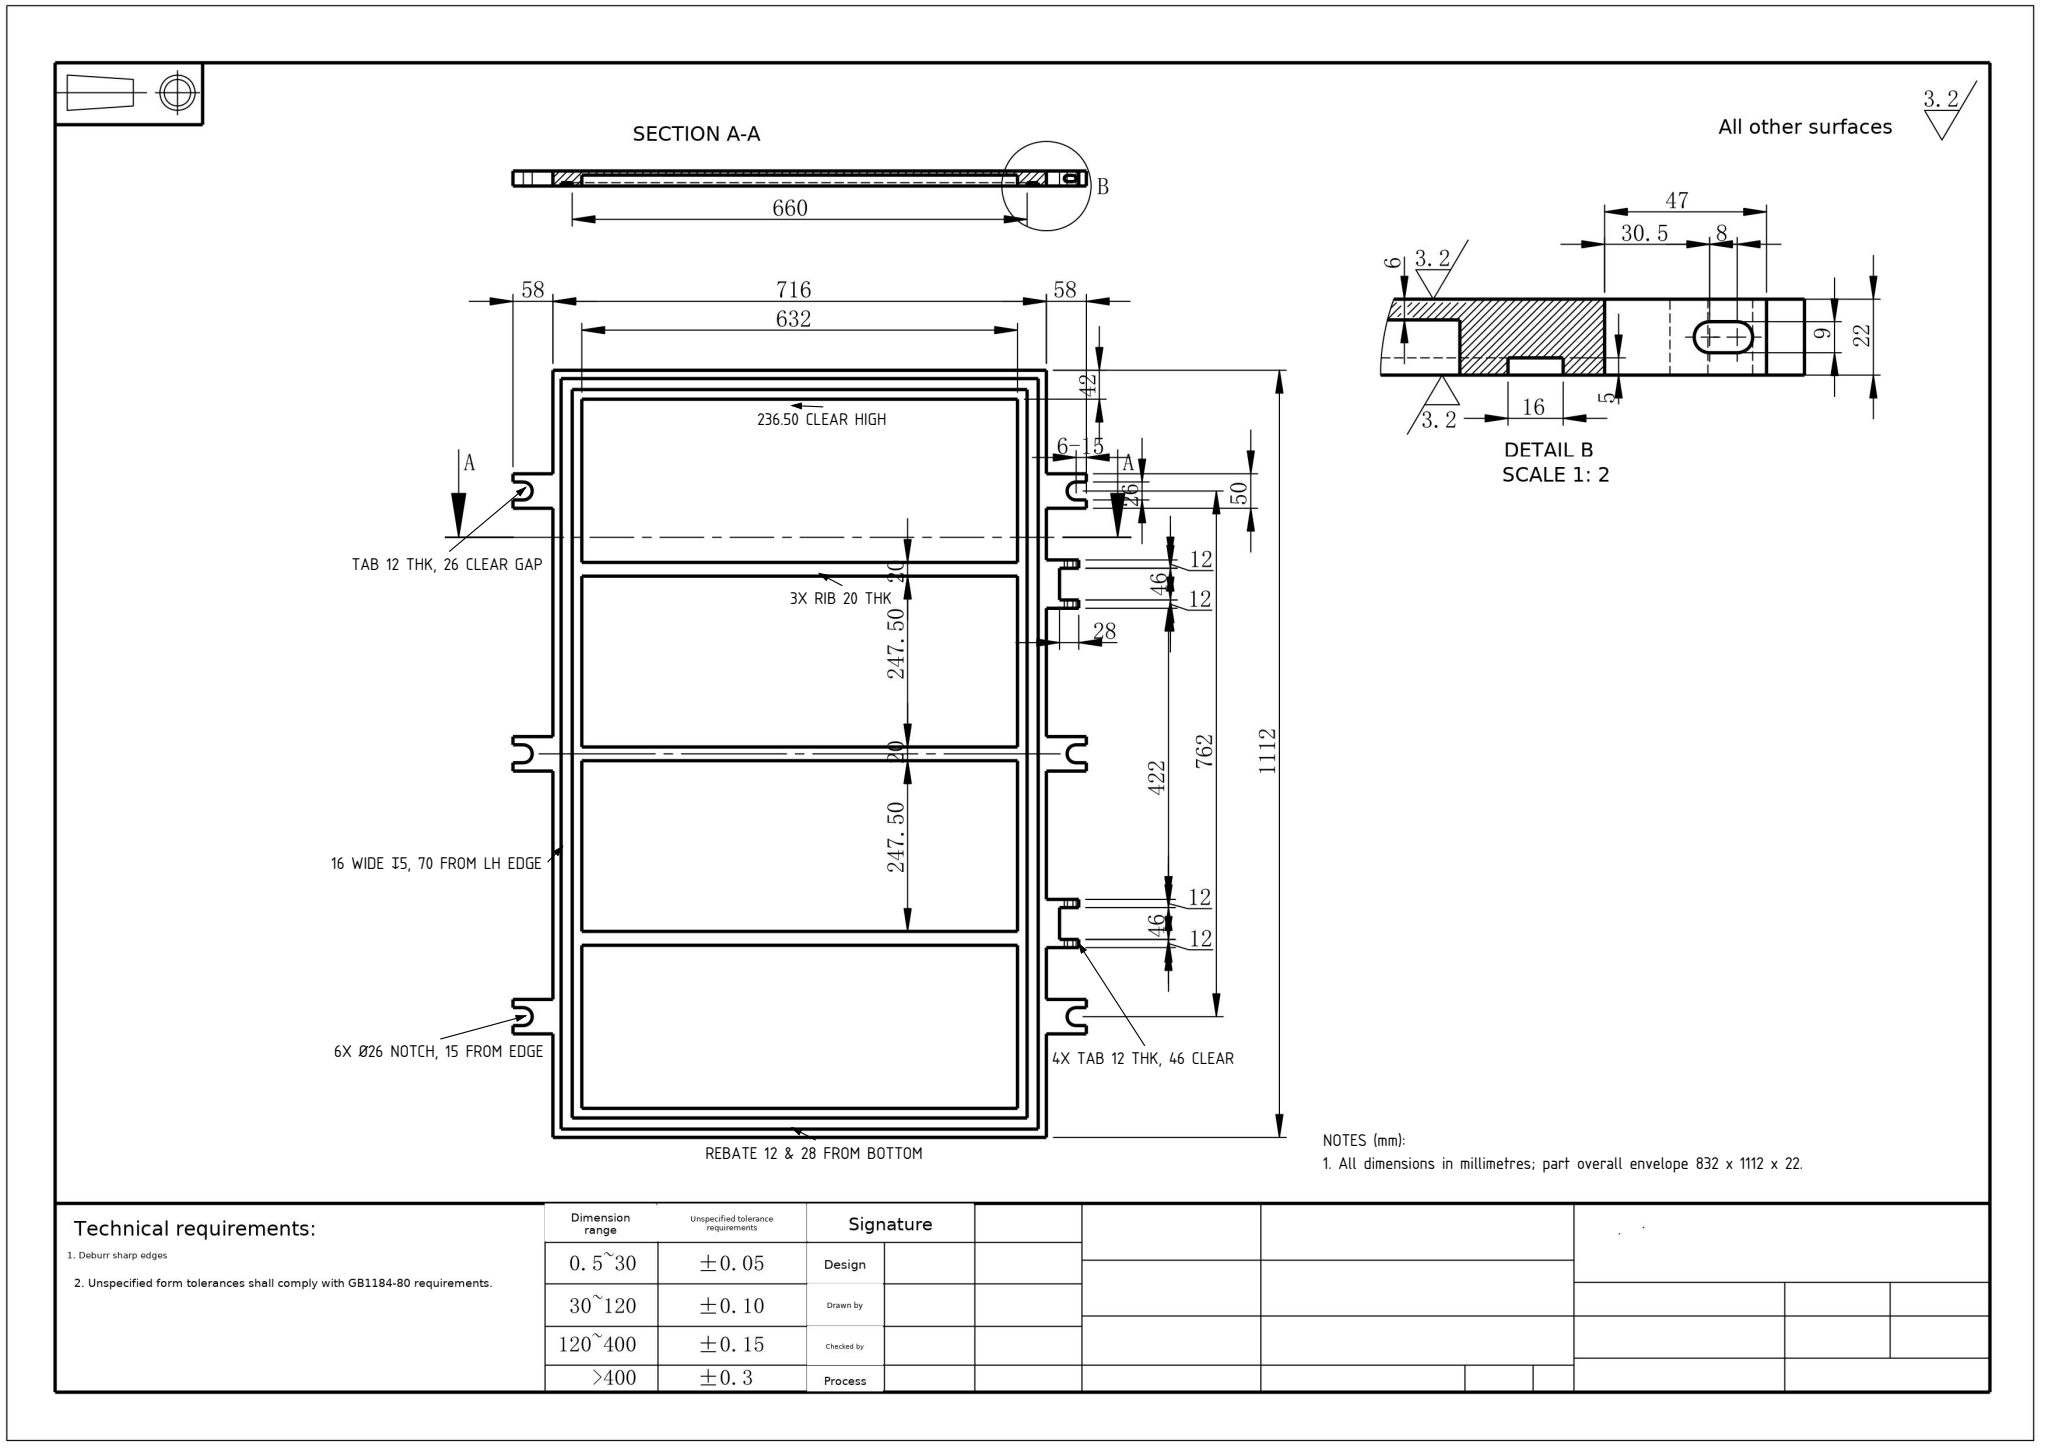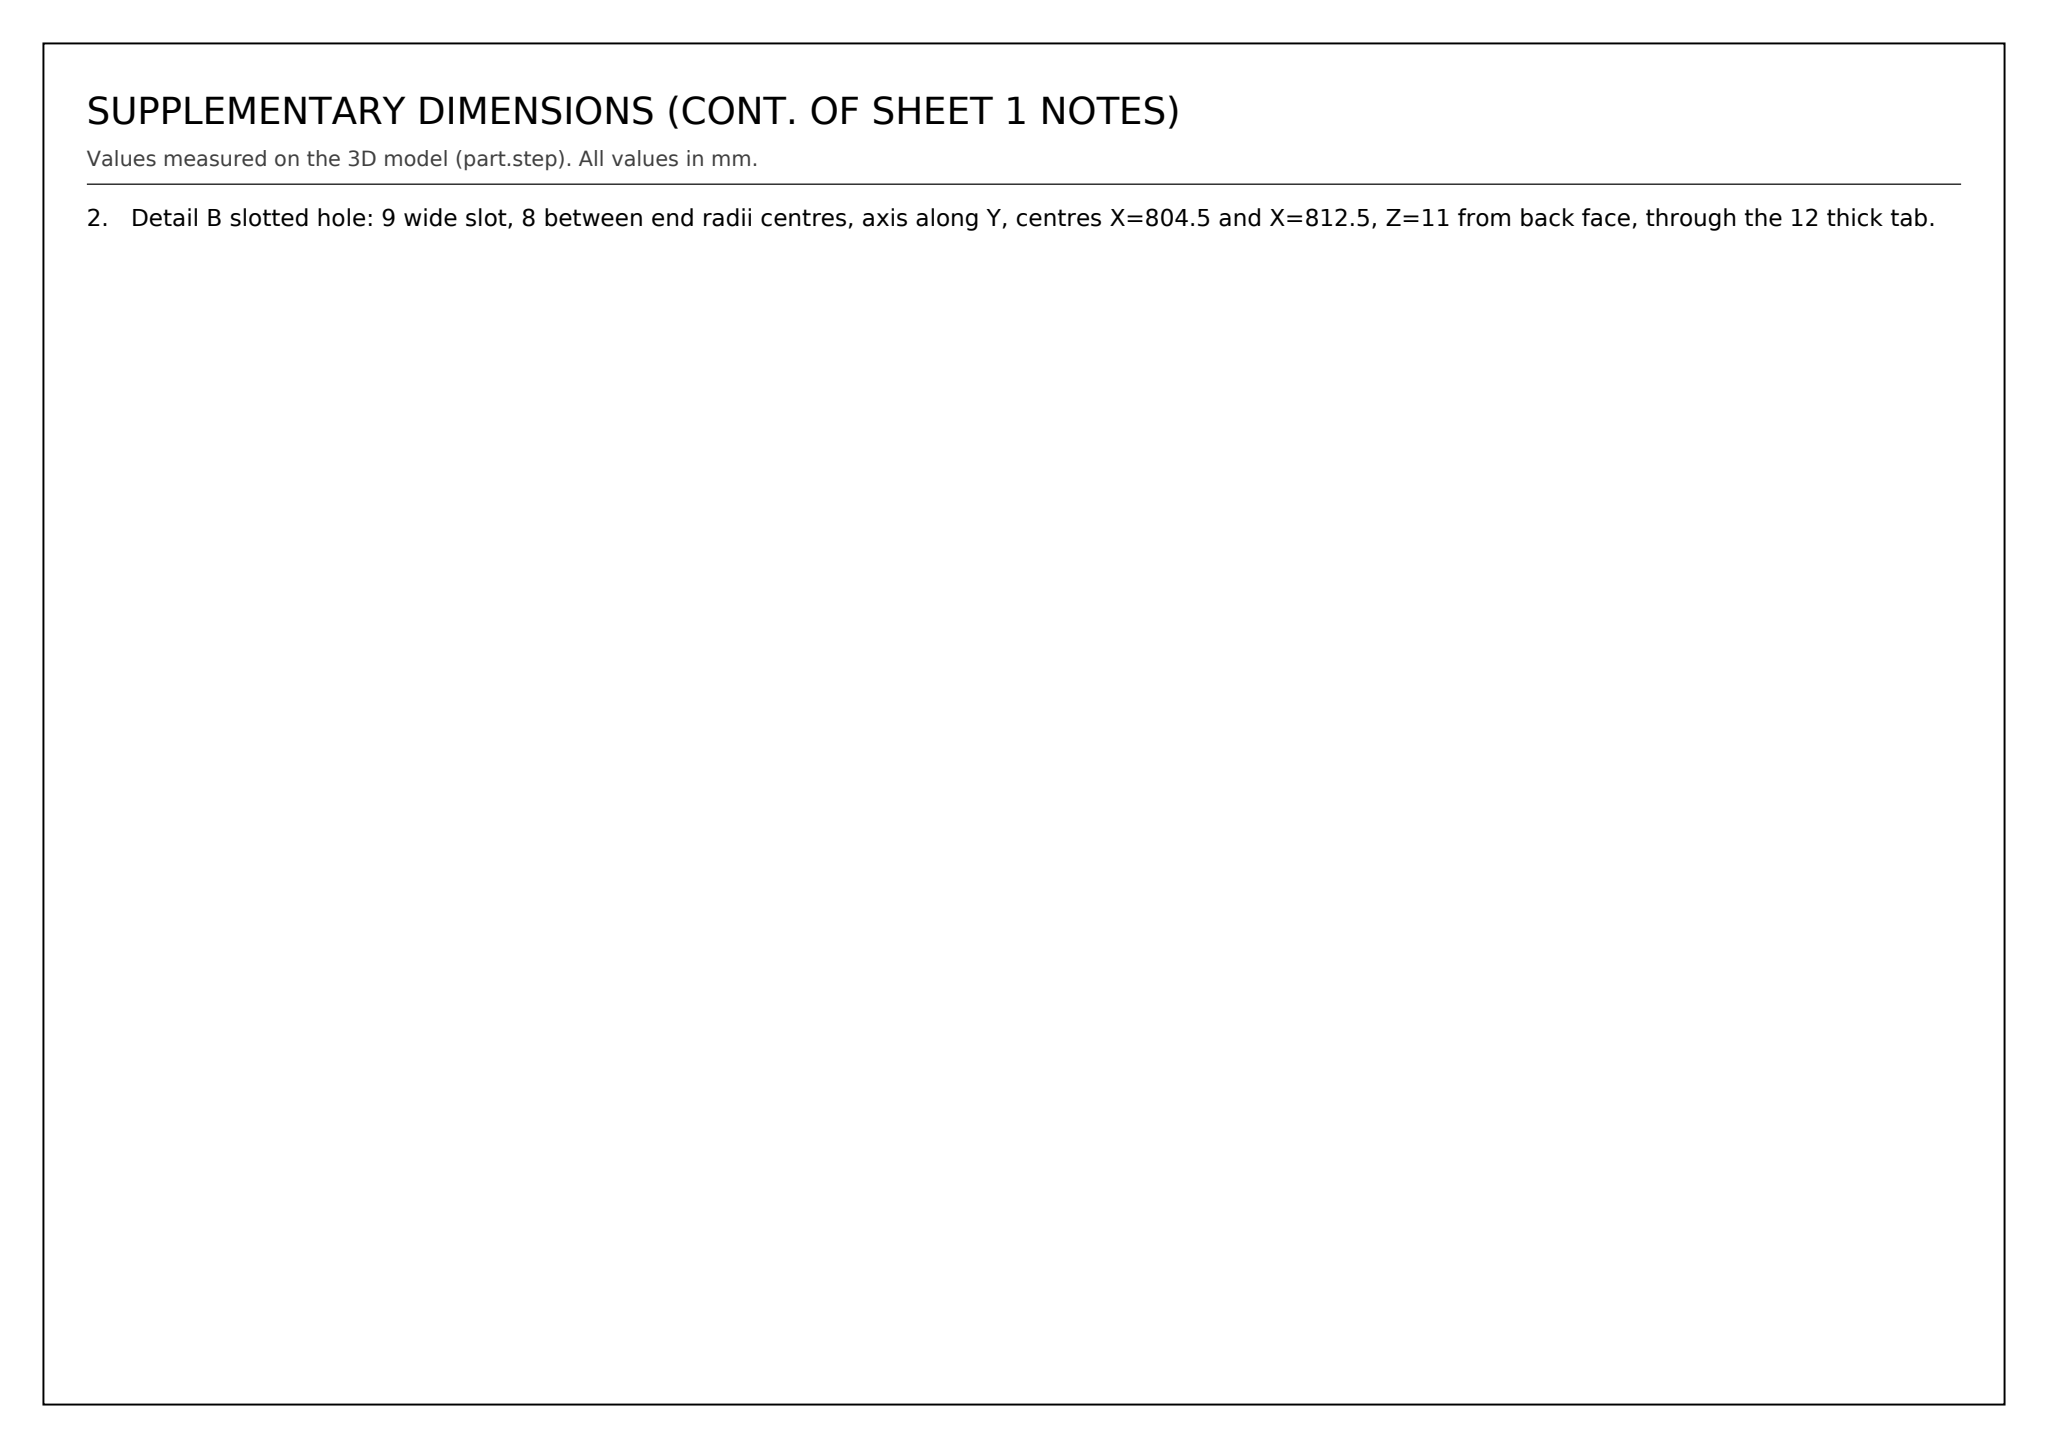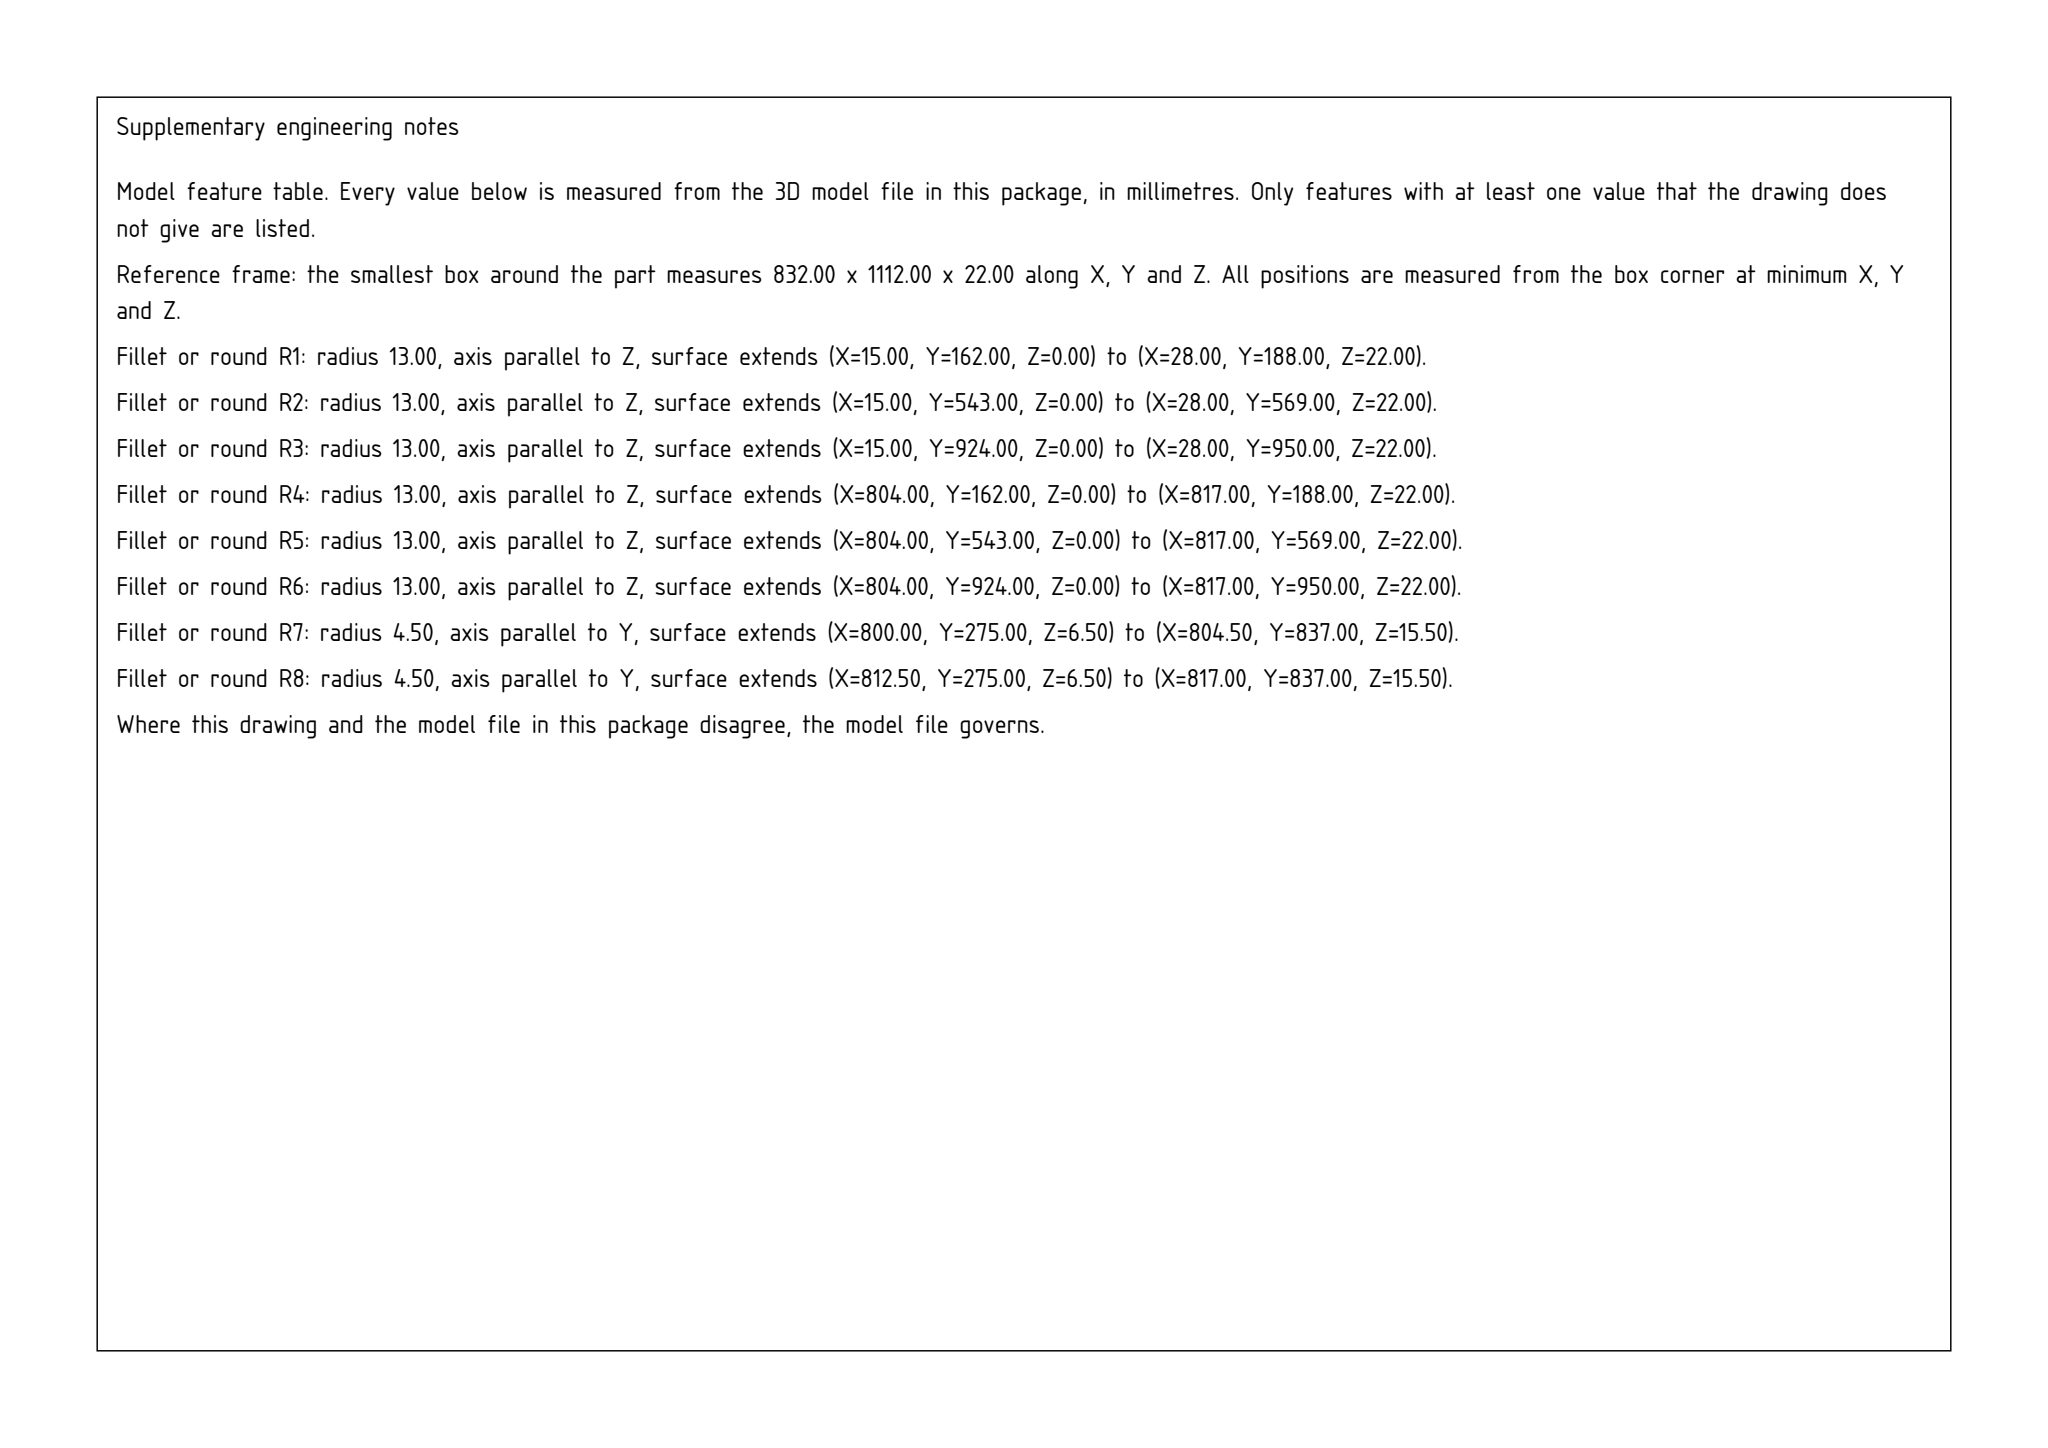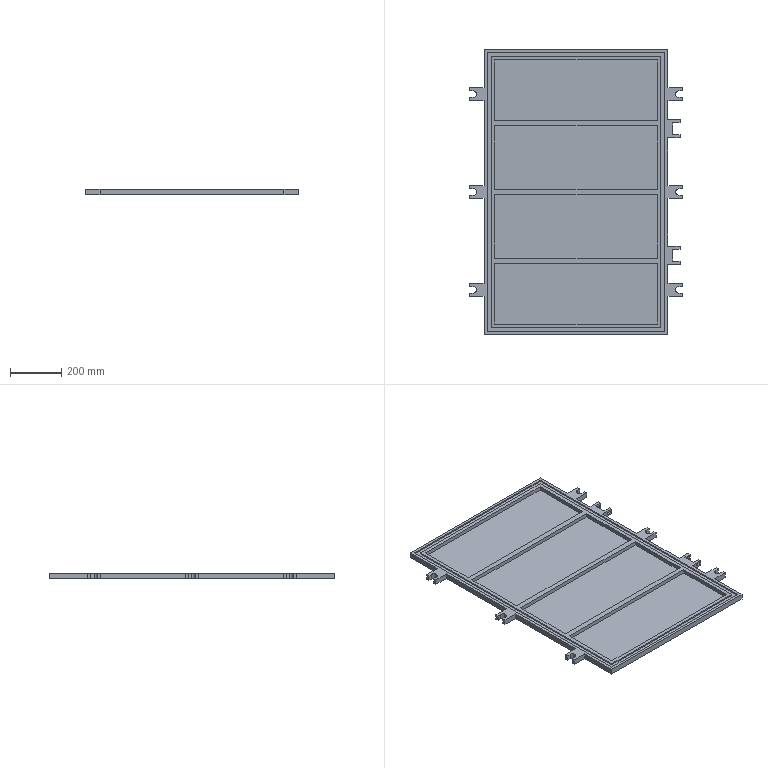Part | SolidWorks | mm | 1 solid | 119 faces | box 832 x 1112 x 22 mm | volume 7825985 mm3 | plane 102 | cylinder 17 | commonest cylinder face diameters 26 x9 9 x8
Drawing notes:
All dimensions in millimetres; part overall envelope 832 x 1112 x 22. | from the solid: bbox_xyz [832.0, 1112.0, 22.0] in mm
Glazing rebate ledge in X: step faces 70 and 86 from left edge; mirrored faces 746 and 762 from left edge (70 and 86 from right edge), ledge 16 wide, 5 deep (Z=17 to 22). | from the solid: axis_planes x=70.0 and x=86.0 (z 17-22), x=746.0 and x=762.0 (z 17-22)
Glazing rebate ledge in Y: step faces 12 and 28 from bottom edge; mirrored faces 1084 and 1100 from bottom edge (28 and 12 from top edge). | from the solid: axis_planes y=12.0 and y=28.0, y=1084.0 and y=1100.0 (z 17-22)
Uppermost and lowermost glazing openings 236.50 clear high: lower Y=42 to Y=278.5, upper Y=833.5 to Y=1070 from bottom edge. | from the solid: axis_planes x=100.0 extents y [42.0, 278.5] and y [833.5, 1070.0]
Horizontal glazing divider ribs 20 thick, 3 places: Y=278.5 to 298.5, Y=546 to 566 and Y=813.5 to 833.5 from bottom edge. | from the solid: axis_planes x=100.0 extents y [42.0,278.5], [298.5,546.0], [566.0,813.5], [833.5,1070.0]
Side slotted tabs 12 thick (4 places): tab faces at Y=275/287 and Y=333/345, mirrored at Y=767/779 and Y=825/837 from bottom edge; 46 clear between each pair. | from the solid: axis_planes y=275.0, y=287.0, y=333.0 (x 793-821); slot cylinders spanning y 275-287, 333-345, 767-779, 825-837
Side edge notch tabs 12 thick with 26 clear gap: faces at Y=162 and Y=188, mirrored at Y=924 and Y=950 from bottom edge. | from the solid: axis_planes y=150.0, 162.0, 188.0, 200.0 (x 0-15 / 817-832) and y=912.0, 924.0, 950.0, 962.0
6X Ø26 half-round edge notch through 22 thk: centres X=15 from left edge and X=817 (15 from right edge), at Y=175, 556 and 937 from bottom edge. | from the solid: cylinders dia 26.0, axis z, at (15,175), (15,556), (15,937), (817,175), (817,556), (817,937), from z=0 to 22, 180 deg
Detail B slotted hole: 9 wide slot, 8 between end radii centres, axis along Y, centres X=804.5 and X=812.5, Z=11 from back face, through the 12 thick tab. | from the solid: cylinders dia 9.0, axis y, at x=804.5 and x=812.5, z=11.0, spans y 275-287, 333-345, 767-779, 825-837
build123d program:
from build123d import *

# Parameters (mm, degrees)
SKETCH1_W               = 716
SKETCH1_H               = 1112
SKETCH1_W_2             = 632
SKETCH1_H_2             = 1028
BOSS_EXTRUDE1_DEPTH     = 22
SKETCH2_W               = 692
SKETCH2_H               = 1088
SKETCH2_W_2             = 660
SKETCH2_H_2             = 1056
CUT_EXTRUDE1_DEPTH      = 5
SKETCH3_W               = 652
SKETCH3_H               = 1048
CUT_EXTRUDE2_DEPTH      = 6
SKETCH4_W               = 652
SKETCH4_H               = 1048
BOSS_EXTRUDE2_DEPTH     = 6
SKETCH5_W               = 632
SKETCH5_H               = 20
BOSS_EXTRUDE3_DEPTH     = 16
LPATTERN1_COUNT         = 2
LPATTERN1_PITCH         = 267.5
LPATTERN1_COL_COUNT     = 2
LPATTERN1_COL_PITCH     = 267.5
SKETCH6_W               = 58
SKETCH6_H               = 50
BOSS_EXTRUDE4_DEPTH     = 22
CUT_EXTRUDE3_DEPTH      = 695.749
LPATTERN2_COUNT         = 2
LPATTERN2_PITCH         = 381
LPATTERN2_COUNT_DIR2    = 2
LPATTERN2_PITCH_DIR2    = 381
MIRROR1_COPY_1_SKETCH_W = 58
MIRROR1_COPY_1_SKETCH_H = 50
MIRROR1_COPY_1_DEPTH    = 22
MIRROR1_COPY_2_SKETCH_W = 58
MIRROR1_COPY_2_SKETCH_H = 50
MIRROR1_COPY_2_DEPTH    = 22
MIRROR1_COPY_3_SKETCH_W = 58
MIRROR1_COPY_3_SKETCH_H = 50
MIRROR1_COPY_3_DEPTH    = 22
MIRROR1_COPY_4_DEPTH    = 695.749
MIRROR1_COPY_5_DEPTH    = 695.749
MIRROR1_COPY_6_DEPTH    = 695.749
SKETCH13_W              = 22
SKETCH13_H              = 70
BOSS_EXTRUDE5_DEPTH     = 47
SKETCH16_W              = 56
SKETCH16_H              = 46
CUT_EXTRUDE6_DEPTH      = 695.749
CUT_EXTRUDE5_REACH      = 936.938
LPATTERN3_COUNT         = 2
LPATTERN3_PITCH         = 492


with BuildPart() as part:
    # Sketch1 → Boss-Extrude1 (new body)
    with BuildSketch(Plane.XY):
        Rectangle(SKETCH1_W, SKETCH1_H)
        Rectangle(SKETCH1_W_2, SKETCH1_H_2, mode=Mode.SUBTRACT)
    extrude(amount=BOSS_EXTRUDE1_DEPTH)

    # Sketch2 → Cut-Extrude1 (cut)
    with BuildSketch(Plane.XY.offset(22)):
        Rectangle(SKETCH2_W, SKETCH2_H)
        Rectangle(SKETCH2_W_2, SKETCH2_H_2, mode=Mode.SUBTRACT)
    extrude(amount=-CUT_EXTRUDE1_DEPTH, mode=Mode.SUBTRACT)

    # Sketch3 → Cut-Extrude2 (cut)
    with BuildSketch(Plane(origin=(0, 0, 0), x_dir=(-1, 0, 0), z_dir=(0, 0, -1))):
        Rectangle(SKETCH3_W, SKETCH3_H)
    extrude(amount=-CUT_EXTRUDE2_DEPTH, mode=Mode.SUBTRACT)


with BuildPart() as body_2:
    # Sketch4 → Boss-Extrude2 (new body)
    with BuildSketch(Plane(origin=(0, 0, 0), x_dir=(-1, 0, 0), z_dir=(0, 0, -1))):
        Rectangle(SKETCH4_W, SKETCH4_H)
    extrude(amount=-BOSS_EXTRUDE2_DEPTH)


with BuildPart() as body_3:
    # Sketch5 → Boss-Extrude3 (new body)
    with BuildSketch(Plane.XY.offset(6)):
        Rectangle(SKETCH5_W, SKETCH5_H)
    boss_extrude3 = extrude(amount=BOSS_EXTRUDE3_DEPTH)


with BuildPart() as part_1:
    add(part.part)

    add(body_2.part)  # LPattern1 merges body 2
    # LPattern1: Boss-Extrude3 ×2
    with Locations(*[(0, i * LPATTERN1_PITCH, 0) for i in range(1, LPATTERN1_COUNT)]):
        add(boss_extrude3)


with BuildPart() as lpattern1_col_1:
    # LPattern1 col: Boss-Extrude3 ×2
    with Locations(*[(0, -i * LPATTERN1_COL_PITCH, 0) for i in range(1, LPATTERN1_COL_COUNT)]):
        add(boss_extrude3)


with BuildPart() as part_2:
    add(part_1.part)

    # LPattern1 col united with what the copie: union body 3, LPattern1 col_1
    add(body_3.part)
    add(lpattern1_col_1.part)

    # Sketch6 → Boss-Extrude4 (add)
    with BuildSketch(Plane.XY.offset(22)):
        with Locations((387, 0)):
            Rectangle(SKETCH6_W, SKETCH6_H)
    boss_extrude4 = extrude(amount=-BOSS_EXTRUDE4_DEPTH)

    # Sketch7 → Cut-Extrude3 (cut, through all)
    with BuildSketch(Plane.XY.offset(22)):
        with BuildLine():
            Line((416, -13), (401, -13))
            ThreePointArc((401, -13), (388, 0), (401, 13))
            Line((401, 13), (416, 13))
            ThreePointArc((416, 13), (429, 0), (416, -13))
        make_face()
    cut_extrude3 = extrude(amount=-CUT_EXTRUDE3_DEPTH, mode=Mode.SUBTRACT)

    # LPattern2: Boss-Extrude4, Cut-Extrude3 2 × 2
    with Locations(*[Vector(0, -1, 0) * (i * LPATTERN2_PITCH) + Vector(0, 1, 0) * (j * LPATTERN2_PITCH_DIR2) for i in range(LPATTERN2_COUNT) for j in range(LPATTERN2_COUNT_DIR2) if (i, j) != (0, 0)]):
        add(boss_extrude4)
        add(cut_extrude3, mode=Mode.SUBTRACT)

    # Mirror1: Boss-Extrude4, Cut-Extrude3 across plane
    add(boss_extrude4.mirror(Plane(origin=(0, 0, 0), x_dir=(0, 0, 1), z_dir=(1, 0, 0))))
    add(cut_extrude3.mirror(Plane(origin=(0, 0, 0), x_dir=(0, 0, 1), z_dir=(1, 0, 0))), mode=Mode.SUBTRACT)

    # Mirror1 copy 1 sketch → Mirror1 copy 1 (add)
    with BuildSketch(Plane(origin=(0, 381, 22), x_dir=(-1, 0, 0), z_dir=(0, 0, 1))):
        with Locations((387, 0)):
            Rectangle(MIRROR1_COPY_1_SKETCH_W, MIRROR1_COPY_1_SKETCH_H)
    extrude(amount=-MIRROR1_COPY_1_DEPTH)

    # Mirror1 copy 2 sketch → Mirror1 copy 2 (add)
    with BuildSketch(Plane(origin=(0, -381, 22), x_dir=(-1, 0, 0), z_dir=(0, 0, 1))):
        with Locations((387, 0)):
            Rectangle(MIRROR1_COPY_2_SKETCH_W, MIRROR1_COPY_2_SKETCH_H)
    extrude(amount=-MIRROR1_COPY_2_DEPTH)

    # Mirror1 copy 3 sketch → Mirror1 copy 3 (add)
    with BuildSketch(Plane(origin=(0, 0, 22), x_dir=(-1, 0, 0), z_dir=(0, 0, 1))):
        with Locations((387, 0)):
            Rectangle(MIRROR1_COPY_3_SKETCH_W, MIRROR1_COPY_3_SKETCH_H)
    extrude(amount=-MIRROR1_COPY_3_DEPTH)

    # Mirror1 copy 4 sketch → Mirror1 copy 4 (cut, through all)
    with BuildSketch(Plane(origin=(0, 381, 22), x_dir=(-1, 0, 0), z_dir=(0, 0, 1))):
        with BuildLine():
            Line((416, 13), (401, 13))
            ThreePointArc((401, 13), (388, 0), (401, -13))
            Line((401, -13), (416, -13))
            ThreePointArc((416, -13), (429, 0), (416, 13))
        make_face()
    extrude(amount=-MIRROR1_COPY_4_DEPTH, mode=Mode.SUBTRACT)

    # Mirror1 copy 5 sketch → Mirror1 copy 5 (cut, through all)
    with BuildSketch(Plane(origin=(0, -381, 22), x_dir=(-1, 0, 0), z_dir=(0, 0, 1))):
        with BuildLine():
            Line((416, 13), (401, 13))
            ThreePointArc((401, 13), (388, 0), (401, -13))
            Line((401, -13), (416, -13))
            ThreePointArc((416, -13), (429, 0), (416, 13))
        make_face()
    extrude(amount=-MIRROR1_COPY_5_DEPTH, mode=Mode.SUBTRACT)

    # Mirror1 copy 6 sketch → Mirror1 copy 6 (cut, through all)
    with BuildSketch(Plane(origin=(0, 0, 22), x_dir=(-1, 0, 0), z_dir=(0, 0, 1))):
        with BuildLine():
            Line((416, 13), (401, 13))
            ThreePointArc((401, 13), (388, 0), (401, -13))
            Line((401, -13), (416, -13))
            ThreePointArc((416, -13), (429, 0), (416, 13))
        make_face()
    extrude(amount=-MIRROR1_COPY_6_DEPTH, mode=Mode.SUBTRACT)

    # Sketch13 → Boss-Extrude5 (add)
    with BuildSketch(Plane(origin=(358, 0, -336), x_dir=(0, 0, -1), z_dir=(1, 0, 0))):
        with Locations((-347, 246)):
            Rectangle(SKETCH13_W, SKETCH13_H)
    boss_extrude5 = extrude(amount=BOSS_EXTRUDE5_DEPTH)

    # Sketch16 → Cut-Extrude6 (cut, through all)
    with BuildSketch(Plane(origin=(0, 0, 0), x_dir=(-1, 0, 0), z_dir=(0, 0, -1))):
        with Locations((-405, 246)):
            Rectangle(SKETCH16_W, SKETCH16_H)
    cut_extrude6 = extrude(amount=-CUT_EXTRUDE6_DEPTH, mode=Mode.SUBTRACT)

    # Cut-Extrude5: up to this face of the body (flat: up to its plane)
    cut_extrude5_end = Plane(part_2.part.faces().sort_by_distance((381.5, 211, 11))[0])
    # Sketch15 → Cut-Extrude5 (cut, up to the picked face)
    with BuildSketch(Plane(origin=(0, 281, 0), x_dir=(1, 0, 0), z_dir=(0, 1, 0)), mode=Mode.PRIVATE) as cut_extrude5_sk1:
        with BuildLine():
            Line((388.5, -6.5), (396.5, -6.5))
            ThreePointArc((396.5, -6.5), (401, -11), (396.5, -15.5))
            Line((396.5, -15.5), (388.5, -15.5))
            ThreePointArc((388.5, -15.5), (384, -11), (388.5, -6.5))
        make_face()
    cut_extrude5_tool1 = split(extrude(cut_extrude5_sk1.sketch, amount=-CUT_EXTRUDE5_REACH, mode=Mode.PRIVATE), bisect_by=cut_extrude5_end, keep=Keep.BOTH, mode=Mode.PRIVATE)
    cut_extrude5 = cut_extrude5_tool1.solids().sort_by(Axis((392.5, 281, 11), (0, -1, 0)))[0]
    add(cut_extrude5, mode=Mode.SUBTRACT)

    # LPattern3: Boss-Extrude5, Cut-Extrude6, Cut-Extrude5 ×2
    with Locations(*[(0, -i * LPATTERN3_PITCH, 0) for i in range(1, LPATTERN3_COUNT)]):
        add(boss_extrude5)
        add(cut_extrude6, mode=Mode.SUBTRACT)
        add(cut_extrude5, mode=Mode.SUBTRACT)


solid = part_2.part